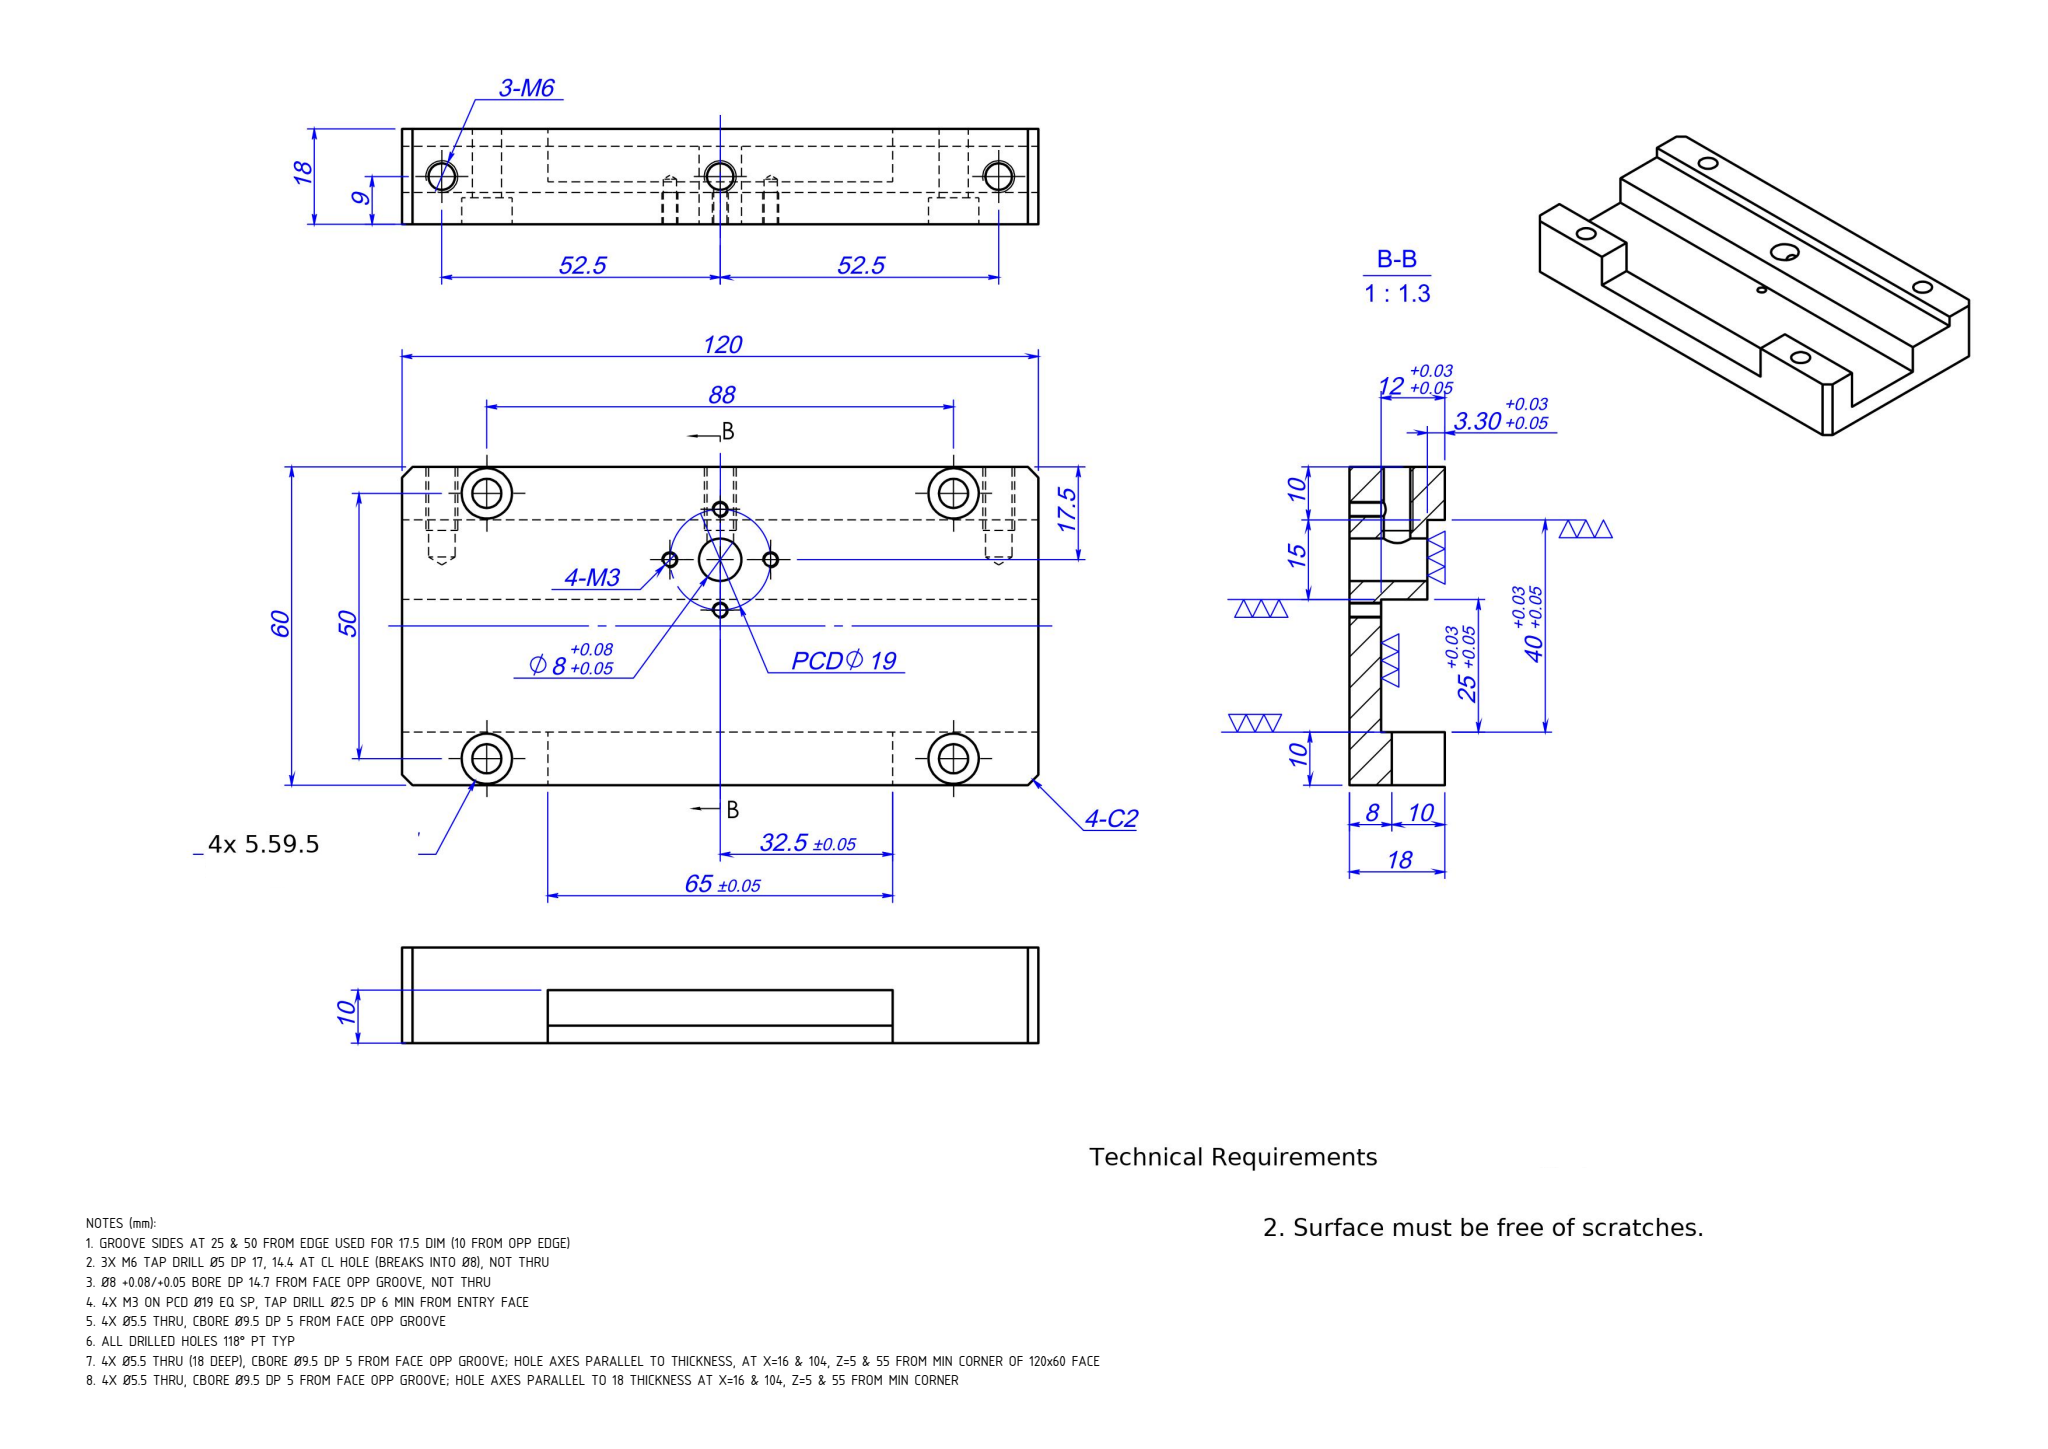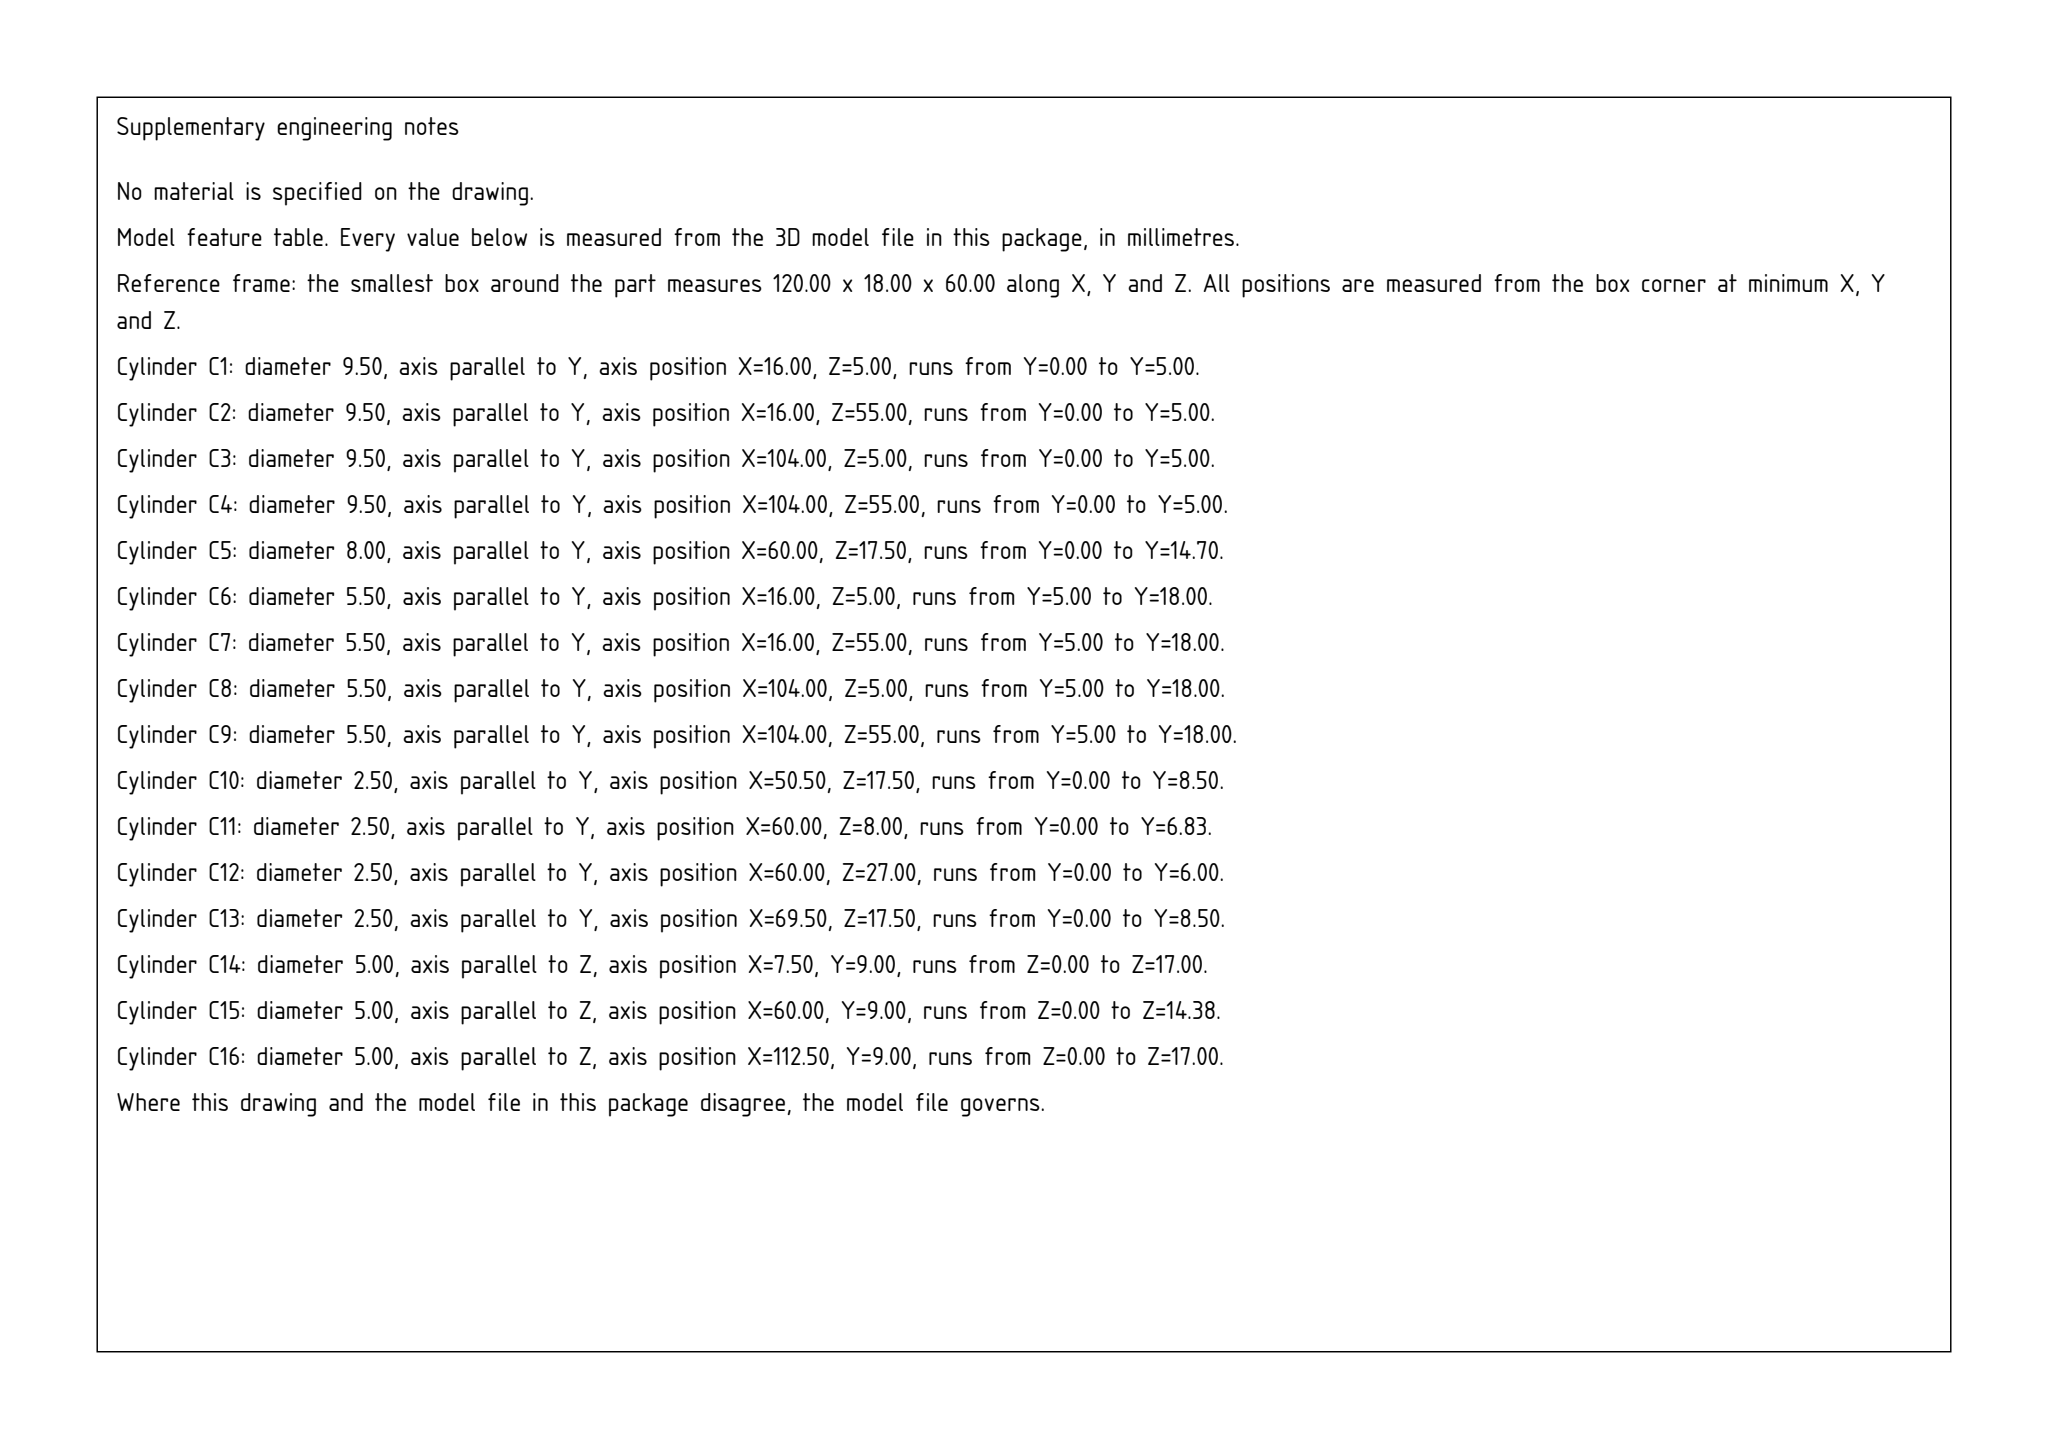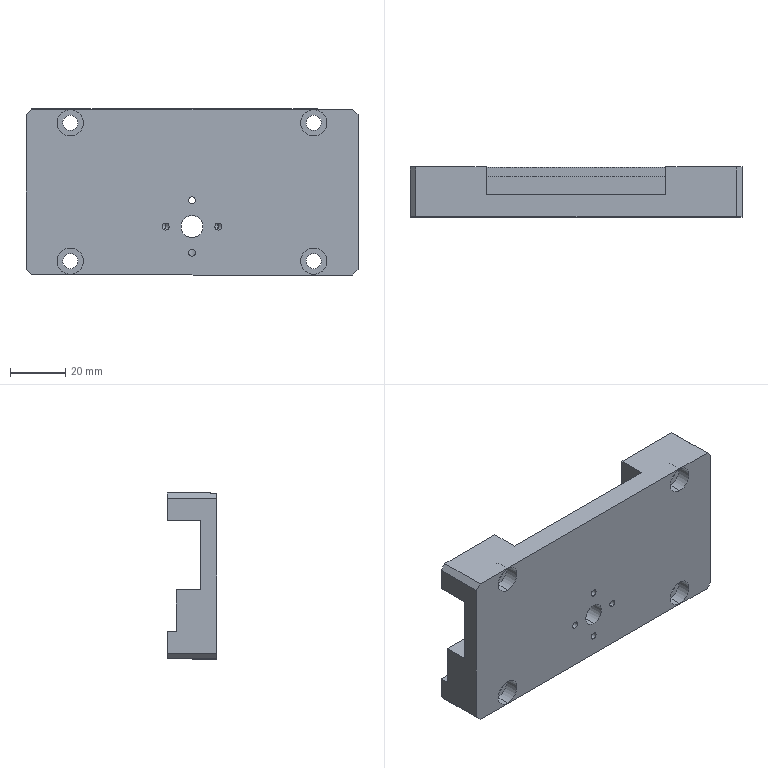Part | SolidWorks | mm | 1 solid | 64 faces | box 120 x 18 x 60 mm | volume 76520 mm3 | cylinder 32 | plane 24 | cone 8 | commonest cylinder face diameters 2.5 x8 5.5 x8 9.5 x8 5 x6 8 x2
Drawing notes:
GROOVE SIDES AT 25 & 50 FROM EDGE USED FOR 17.5 DIM (10 FROM OPP EDGE) | from the solid: z-planes 25.0 & 50.0 in bbox z=60; hole CL z=17.5 fixes datum edge z=0
3X M6 TAP DRILL Ø5 DP 17, 14.4 AT CL HOLE (BREAKS INTO Ø8), NOT THRU | from the solid: cyl Ø5 axis z L17 at (7.5,9) & (112.5,9); Ø5 axis z L14.38 at (60,9); part z=60
Ø8 +0.08/+0.05 BORE DP 14.7 FROM FACE OPP GROOVE, NOT THRU | from the solid: cyl Ø8 axis y L14.7 at (60,17.5); y-plane 14.7 vs top y=18, thk 18
4X M3 ON PCD Ø19 EQ SP, TAP DRILL Ø2.5 DP 6 MIN FROM ENTRY FACE | from the solid: Ø2.5 axis y at (50.5,17.5) & (69.5,17.5) L8.5; (60,8) L6.84; (60,27) L6.0
4X Ø5.5 THRU, CBORE Ø9.5 DP 5 FROM FACE OPP GROOVE | from the solid: Ø5.5 axis y L13 at (16/104, 5/55) + Ø9.5 axis y L5 same XZ; y-planes 5.0 x4; 13+5=18
ALL DRILLED HOLES 118° PT TYP | from the solid: cones 118° ref dia 2.5 (x4) and 5.0 (x4)
4X Ø5.5 THRU (18 DEEP), CBORE Ø9.5 DP 5 FROM FACE OPP GROOVE; HOLE AXES PARALLEL TO THICKNESS, AT X=16 & 104, Z=5 & 55 FROM MIN CORNER OF 120x60 FACE | from the solid: cylinders [5.5,'y',[16/104,null,5/55],13] and [9.5,'y',[16/104,null,5/55],5]; bbox_xyz 120x18x60
4X Ø5.5 THRU, CBORE Ø9.5 DP 5 FROM FACE OPP GROOVE; HOLE AXES PARALLEL TO 18 THICKNESS AT X=16 & 104, Z=5 & 55 FROM MIN CORNER | from the solid: cylinders [5.5,"y",[16/104,null,5/55],13.0] and [9.5,"y",[16/104,null,5/55],5.0]
build123d program:
from build123d import *

# Parameters (mm, degrees)
SKETCH1_W                                            = 120
SKETCH1_H                                            = 60
EXTRUDE1_DEPTH                                       = 14.7
SKETCH4_W                                            = 120
SKETCH4_H                                            = 10
EXTRUDE3_DEPTH                                       = 3.3
SKETCH2_R                                            = 4
CUT_EXTRUDE1_DEPTH                                   = 69.674
SKETCH3_W                                            = 120
SKETCH3_H                                            = 25
CUT_EXTRUDE2_DEPTH                                   = 8.7
SKETCH5_W                                            = 65
SKETCH5_H                                            = 10
CUT_EXTRUDE3_DEPTH                                   = 10
M6_TAPPED_HOLE1_D                                    = 5
M6_TAPPED_HOLE1_DEPTH                                = 17
M6_TAPPED_HOLE1_TIP                                  = 1.502
COUNTERBORE_FOR_M5_HEX_SOCKET_HEAD_CAP_S_D           = 5.5
COUNTERBORE_FOR_M5_HEX_SOCKET_HEAD_CAP_S_CBORE_D     = 9.5
COUNTERBORE_FOR_M5_HEX_SOCKET_HEAD_CAP_S_CBORE_DEPTH = 5
M3_TAPPED_HOLE1_D                                    = 2.5
M3_TAPPED_HOLE1_DEPTH                                = 8.5
M3_TAPPED_HOLE1_TIP                                  = 0.7511
CHAMFER1_SIZE                                        = 2


with BuildPart() as part:
    # Sketch1 → Extrude1 (new body)
    with BuildSketch(Plane(origin=(0, 0, 0), x_dir=(1, 0, 0), z_dir=(0, 1, 0))):
        Rectangle(SKETCH1_W, SKETCH1_H)
    extrude(amount=EXTRUDE1_DEPTH)

    # Sketch4 → Extrude3 (add)
    with BuildSketch(Plane(origin=(0, 14.7, 0), x_dir=(1, 0, 0), z_dir=(0, 1, 0))):
        with Locations((0, -25)):
            Rectangle(SKETCH4_W, SKETCH4_H)
        with Locations((0, 25)):
            Rectangle(SKETCH4_W, SKETCH4_H)
    extrude(amount=EXTRUDE3_DEPTH)

    # Sketch2 → Cut-Extrude1 (cut, through all)
    with BuildSketch(Plane(origin=(0, 14.7, 0), x_dir=(1, 0, 0), z_dir=(0, 1, 0))):
        with Locations(Location((0, 12.5, 0), (0, 0, 270))):
            Circle(SKETCH2_R)
    extrude(amount=-CUT_EXTRUDE1_DEPTH, mode=Mode.SUBTRACT)

    # Sketch3 → Cut-Extrude2 (cut)
    with BuildSketch(Plane(origin=(0, 14.7, 0), x_dir=(1, 0, 0), z_dir=(0, 1, 0))):
        with Locations((0, -7.5)):
            Rectangle(SKETCH3_W, SKETCH3_H)
    extrude(amount=-CUT_EXTRUDE2_DEPTH, mode=Mode.SUBTRACT)

    # Sketch5 → Cut-Extrude3 (cut)
    with BuildSketch(Plane(origin=(0, 18, 0), x_dir=(1, 0, 0), z_dir=(0, 1, 0))):
        with Locations((0, -25)):
            Rectangle(SKETCH5_W, SKETCH5_H)
    extrude(amount=-CUT_EXTRUDE3_DEPTH, mode=Mode.SUBTRACT)

    # M6 Tapped Hole1
    with Locations(Plane(origin=(0, 0, -30), x_dir=(-1, 0, 0), z_dir=(0, 0, -1))):
        with Locations((0, 9), (-52.5, 9), (52.5, 9)):
            Hole(M6_TAPPED_HOLE1_D / 2, depth=M6_TAPPED_HOLE1_DEPTH)
            with Locations((0, 0, -(M6_TAPPED_HOLE1_DEPTH + M6_TAPPED_HOLE1_TIP / 2))):  # 118° drill point
                Cone(0, M6_TAPPED_HOLE1_D / 2, M6_TAPPED_HOLE1_TIP, mode=Mode.SUBTRACT)

    # Counterbore for M5 Hex Socket Head Cap S (through all)
    with Locations(Plane.XZ):
        with Locations((-44, -25), (-44, 25), (44, 25), (44, -25)):
            CounterBoreHole(COUNTERBORE_FOR_M5_HEX_SOCKET_HEAD_CAP_S_D / 2, COUNTERBORE_FOR_M5_HEX_SOCKET_HEAD_CAP_S_CBORE_D / 2, COUNTERBORE_FOR_M5_HEX_SOCKET_HEAD_CAP_S_CBORE_DEPTH)

    # M3 Tapped Hole1
    with Locations(Plane.XZ):
        with Locations((0, -3), (9.5, -12.5), (0, -22), (-9.5, -12.5)):
            Hole(M3_TAPPED_HOLE1_D / 2, depth=M3_TAPPED_HOLE1_DEPTH)
            with Locations((0, 0, -(M3_TAPPED_HOLE1_DEPTH + M3_TAPPED_HOLE1_TIP / 2))):  # 118° drill point
                Cone(0, M3_TAPPED_HOLE1_D / 2, M3_TAPPED_HOLE1_TIP, mode=Mode.SUBTRACT)

    # Chamfer1
    chamfer1_edges = [part.edges().sort_by_distance(p)[0] for p in [
        (-60, 9, -30),
        (60, 9, -30),
        (60, 9, 30),
        (-60, 9, 30),
    ]]
    chamfer(chamfer1_edges, length=CHAMFER1_SIZE)


solid = part.part